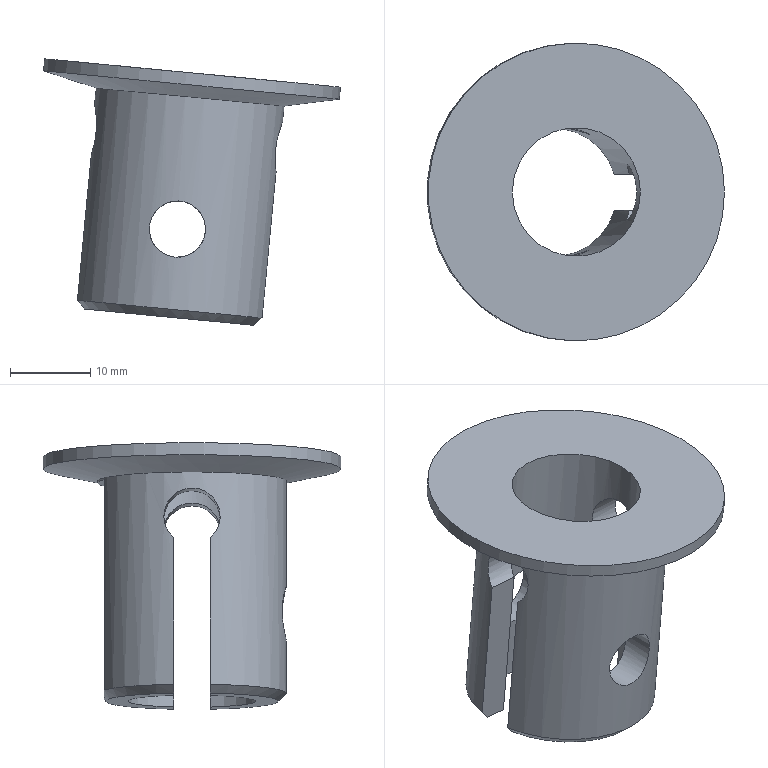Component | NX | XIANWEITAO | 1 solid | 19 faces | volume 7145 mm3 | plane 9 | cylinder 7 | cone 3 | commonest cylinder face diameters 7 x4 16 x1 23.5 x1 37 x1